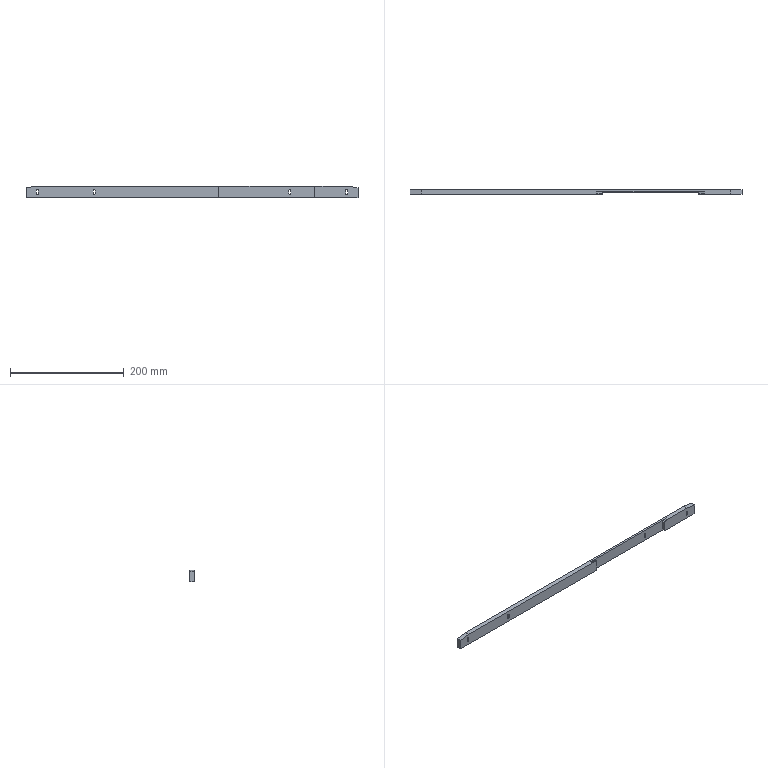Component | SolidWorks | SL010-LeftStreamline-1-1_SL010-02047858StopBarNo.4-1-2 | 1 solid | 32 faces | box 584 x 8 x 21 mm | volume 82637 mm3 | plane 24 | cylinder 8 | commonest cylinder face diameters 3.2 x8 | material White POM
build123d program:
from build123d import *

# Parameters (mm, degrees)
SKETCH1_2_W          = 584
SKETCH1_2_H          = 21
BOSS_EXTRUDE1_DEPTH  = 8
CUT_EXTRUDE1_2_DEPTH = 293.298
CHAMFER1_SIZE        = 3
CHAMFER1_SIZE2       = 20
CHAMFER2_SIZE        = 20
CHAMFER2_SIZE2       = 3
SKETCH4_W            = 169.5
SKETCH4_H            = 3.139
CUT_EXTRUDE3_DEPTH   = 293.863
CHAMFER3_SIZE        = 10
CHAMFER3_SIZE2       = 2.679
SKETCH1_W            = 169.5
SKETCH1_H            = 1.7
CUT_EXTRUDE1_DEPTH   = 293.863


with BuildPart() as part:
    # Sketch1_2 → Boss-Extrude1 (new body)
    with BuildSketch(Plane.XY):
        Rectangle(SKETCH1_2_W, SKETCH1_2_H)
    extrude(amount=BOSS_EXTRUDE1_DEPTH)

    # Sketch2 → Cut-Extrude1_2 (cut, through all)
    with BuildSketch(Plane.XY.offset(8)):
        with BuildLine():
            Line((173.6, 2.5), (173.6, -2.5))
            ThreePointArc((173.6, -2.5), (172, -4.1), (170.4, -2.5))
            Line((170.4, -2.5), (170.4, 2.5))
            ThreePointArc((170.4, 2.5), (172, 4.1), (173.6, 2.5))
        make_face()
        with BuildLine():
            Line((-273.6, 2.5), (-273.6, -2.5))
            ThreePointArc((-273.6, -2.5), (-272, -4.1), (-270.4, -2.5))
            Line((-270.4, -2.5), (-270.4, 2.5))
            ThreePointArc((-270.4, 2.5), (-272, 4.1), (-273.6, 2.5))
        make_face()
        with BuildLine():
            Line((273.6, 2.5), (273.6, -2.5))
            ThreePointArc((273.6, -2.5), (272, -4.1), (270.4, -2.5))
            Line((270.4, -2.5), (270.4, 2.5))
            ThreePointArc((270.4, 2.5), (272, 4.1), (273.6, 2.5))
        make_face()
        with BuildLine():
            Line((-173.6, 2.5), (-173.6, -2.5))
            ThreePointArc((-173.6, -2.5), (-172, -4.1), (-170.4, -2.5))
            Line((-170.4, -2.5), (-170.4, 2.5))
            ThreePointArc((-170.4, 2.5), (-172, 4.1), (-173.6, 2.5))
        make_face()
    extrude(amount=-CUT_EXTRUDE1_2_DEPTH, mode=Mode.SUBTRACT)

    # Chamfer1
    chamfer1_edges = [part.edges().sort_by_distance(p)[0] for p in [
        (292, 10.5, 4),
    ]]
    chamfer1_side = [part.faces().sort_by_distance(p)[0] for p in [
        (292, 0, 4),
    ]]
    chamfer(chamfer1_edges, length=CHAMFER1_SIZE, length2=CHAMFER1_SIZE2, reference=chamfer1_side[0])

    # Chamfer2
    chamfer2_edges = [part.edges().sort_by_distance(p)[0] for p in [
        (-292, 10.5, 4),
    ]]
    chamfer2_side = [part.faces().sort_by_distance(p)[0] for p in [
        (-10, 10.5, 4),
    ]]
    chamfer(chamfer2_edges, length=CHAMFER2_SIZE, length2=CHAMFER2_SIZE2, reference=chamfer2_side[0])

    # Sketch4 → Cut-Extrude3 (cut, through all)
    with BuildSketch(Plane.XZ.offset(10.5)):
        with Locations((-131.25, 2.431)):
            Rectangle(SKETCH4_W, SKETCH4_H)
    extrude(amount=-CUT_EXTRUDE3_DEPTH, mode=Mode.SUBTRACT)

    # Chamfer3
    chamfer3_edges = [part.edges().sort_by_distance(p)[0] for p in [
        (-216, 10.5, 2.431),
        (-46.5, 10.5, 2.431),
    ]]
    chamfer3_side = [part.faces().sort_by_distance(p)[0] for p in [
        (18.28, 10.5, 4.219),
    ]]
    chamfer(chamfer3_edges, length=CHAMFER3_SIZE, length2=CHAMFER3_SIZE2, reference=chamfer3_side[0])

    # Sketch1 → Cut-Extrude1 (cut, through all)
    with BuildSketch(Plane.XZ.offset(10.5)):
        with Locations((-131.25, 0.35)):
            Rectangle(SKETCH1_W, SKETCH1_H)
    extrude(amount=-CUT_EXTRUDE1_DEPTH, mode=Mode.SUBTRACT)


solid = part.part

# Placed as in the assembly
solid = solid.moved(Location((0, -109.904, -647.535), (-90, 0, 180)))
STEP:
#1=COLOUR_RGB('',0.7922,0.8196,0.9333);
#2=FILL_AREA_STYLE_COLOUR('',#1);
#3=FILL_AREA_STYLE('',(#2));
#4=SURFACE_STYLE_FILL_AREA(#3);
#5=SURFACE_SIDE_STYLE('',(#4));
#6=SURFACE_STYLE_USAGE(.BOTH.,#5);
#7=PRESENTATION_STYLE_ASSIGNMENT((#6));
#8=CARTESIAN_POINT('',(1.831,-4.327,-25.907));
#9=VERTEX_POINT('',#8);
#10=CARTESIAN_POINT('',(1.831,-4.169,-25.907));
#11=VERTEX_POINT('',#10);
#12=CARTESIAN_POINT('',(1.831,-4.293,-25.907));
#13=DIRECTION('',(0.,1.,0.));
#14=VECTOR('',#13,39.37);
#15=LINE('',#12,#14);
#16=EDGE_CURVE('',#9,#11,#15,.T.);
#17=ORIENTED_EDGE('',*,*,#16,.F.);
#18=CARTESIAN_POINT('',(-11.496,-4.327,-25.907));
#19=VERTEX_POINT('',#18);
#20=CARTESIAN_POINT('',(11.496,-4.327,-25.907));
#21=DIRECTION('',(-1.,0.,-0.));
#22=VECTOR('',#21,39.37);
#23=LINE('',#20,#22);
#24=EDGE_CURVE('',#9,#19,#23,.T.);
#25=ORIENTED_EDGE('',*,*,#24,.T.);
#26=CARTESIAN_POINT('',(-11.496,-4.012,-25.907));
#27=VERTEX_POINT('',#26);
#28=CARTESIAN_POINT('',(-11.496,-4.012,-25.907));
#29=DIRECTION('',(-0.,-1.,-0.));
#30=VECTOR('',#29,39.37);
#31=LINE('',#28,#30);
#32=EDGE_CURVE('',#27,#19,#31,.T.);
#33=ORIENTED_EDGE('',*,*,#32,.F.);
#34=CARTESIAN_POINT('',(11.496,-4.012,-25.907));
#35=VERTEX_POINT('',#34);
#36=CARTESIAN_POINT('',(11.496,-4.012,-25.907));
#37=DIRECTION('',(-1.,0.,-0.));
#38=VECTOR('',#37,39.37);
#39=LINE('',#36,#38);
#40=EDGE_CURVE('',#35,#27,#39,.T.);
#41=ORIENTED_EDGE('',*,*,#40,.F.);
#42=CARTESIAN_POINT('',(11.496,-4.327,-25.907));
#43=VERTEX_POINT('',#42);
#44=CARTESIAN_POINT('',(11.496,-4.012,-25.907));
#45=DIRECTION('',(-0.,-1.,-0.));
#46=VECTOR('',#45,39.37);
#47=LINE('',#44,#46);
#48=EDGE_CURVE('',#35,#43,#47,.T.);
#49=ORIENTED_EDGE('',*,*,#48,.T.);
#50=CARTESIAN_POINT('',(8.504,-4.327,-25.907));
#51=VERTEX_POINT('',#50);
#52=CARTESIAN_POINT('',(11.496,-4.327,-25.907));
#53=DIRECTION('',(-1.,0.,-0.));
#54=VECTOR('',#53,39.37);
#55=LINE('',#52,#54);
#56=EDGE_CURVE('',#43,#51,#55,.T.);
#57=ORIENTED_EDGE('',*,*,#56,.T.);
#58=CARTESIAN_POINT('',(8.504,-4.169,-25.907));
#59=VERTEX_POINT('',#58);
#60=CARTESIAN_POINT('',(8.504,-4.293,-25.907));
#61=DIRECTION('',(-0.,-1.,-0.));
#62=VECTOR('',#61,39.37);
#63=LINE('',#60,#62);
#64=EDGE_CURVE('',#59,#51,#63,.T.);
#65=ORIENTED_EDGE('',*,*,#64,.F.);
#66=CARTESIAN_POINT('',(1.831,-4.169,-25.907));
#67=DIRECTION('',(1.,-0.,0.));
#68=VECTOR('',#67,39.37);
#69=LINE('',#66,#68);
#70=EDGE_CURVE('',#11,#59,#69,.T.);
#71=ORIENTED_EDGE('',*,*,#70,.F.);
#72=EDGE_LOOP('',(#17,#25,#33,#41,#49,#57,#65,#71));
#73=FACE_OUTER_BOUND('',#72,.T.);
#74=CARTESIAN_POINT('',(11.496,-4.012,-25.907));
#75=DIRECTION('',(-0.,-0.,1.));
#76=DIRECTION('',(0.,1.,0.));
#77=AXIS2_PLACEMENT_3D('',#74,#75,#76);
#78=PLANE('',#77);
#79=ADVANCED_FACE('',(#73),#78,.F.);
#80=CARTESIAN_POINT('',(-6.835,-4.327,-25.592));
#81=VERTEX_POINT('',#80);
#82=CARTESIAN_POINT('',(-6.835,-4.327,-25.395));
#83=VERTEX_POINT('',#82);
#84=CARTESIAN_POINT('',(-6.835,-4.327,-25.395));
#85=DIRECTION('',(-0.,-0.,1.));
#86=VECTOR('',#85,39.37);
#87=LINE('',#84,#86);
#88=EDGE_CURVE('',#81,#83,#87,.T.);
#89=ORIENTED_EDGE('',*,*,#88,.T.);
#90=CARTESIAN_POINT('',(-6.709,-4.327,-25.395));
#91=VERTEX_POINT('',#90);
#92=CARTESIAN_POINT('',(-6.772,-4.327,-25.395));
#93=DIRECTION('',(0.,1.,0.));
#94=DIRECTION('',(-1.,0.,0.));
#95=AXIS2_PLACEMENT_3D('',#92,#93,#94);
#96=CIRCLE('',#95,0.06299);
#97=EDGE_CURVE('',#83,#91,#96,.T.);
#98=ORIENTED_EDGE('',*,*,#97,.T.);
#99=CARTESIAN_POINT('',(-6.709,-4.327,-25.592));
#100=VERTEX_POINT('',#99);
#101=CARTESIAN_POINT('',(-6.709,-4.327,-25.395));
#102=DIRECTION('',(0.,0.,-1.));
#103=VECTOR('',#102,39.37);
#104=LINE('',#101,#103);
#105=EDGE_CURVE('',#91,#100,#104,.T.);
#106=ORIENTED_EDGE('',*,*,#105,.T.);
#107=CARTESIAN_POINT('',(-6.772,-4.327,-25.592));
#108=DIRECTION('',(0.,1.,0.));
#109=DIRECTION('',(-1.,0.,0.));
#110=AXIS2_PLACEMENT_3D('',#107,#108,#109);
#111=CIRCLE('',#110,0.06299);
#112=EDGE_CURVE('',#100,#81,#111,.T.);
#113=ORIENTED_EDGE('',*,*,#112,.T.);
#114=EDGE_LOOP('',(#89,#98,#106,#113));
#115=FACE_BOUND('',#114,.T.);
#116=CARTESIAN_POINT('',(-10.772,-4.327,-25.592));
#117=VERTEX_POINT('',#116);
#118=CARTESIAN_POINT('',(-10.772,-4.327,-25.395));
#119=VERTEX_POINT('',#118);
#120=CARTESIAN_POINT('',(-10.772,-4.327,-25.395));
#121=DIRECTION('',(-0.,-0.,1.));
#122=VECTOR('',#121,39.37);
#123=LINE('',#120,#122);
#124=EDGE_CURVE('',#117,#119,#123,.T.);
#125=ORIENTED_EDGE('',*,*,#124,.T.);
#126=CARTESIAN_POINT('',(-10.646,-4.327,-25.395));
#127=VERTEX_POINT('',#126);
#128=CARTESIAN_POINT('',(-10.709,-4.327,-25.395));
#129=DIRECTION('',(0.,1.,0.));
#130=DIRECTION('',(-1.,0.,0.));
#131=AXIS2_PLACEMENT_3D('',#128,#129,#130);
#132=CIRCLE('',#131,0.06299);
#133=EDGE_CURVE('',#119,#127,#132,.T.);
#134=ORIENTED_EDGE('',*,*,#133,.T.);
#135=CARTESIAN_POINT('',(-10.646,-4.327,-25.592));
#136=VERTEX_POINT('',#135);
#137=CARTESIAN_POINT('',(-10.646,-4.327,-25.395));
#138=DIRECTION('',(0.,0.,-1.));
#139=VECTOR('',#138,39.37);
#140=LINE('',#137,#139);
#141=EDGE_CURVE('',#127,#136,#140,.T.);
#142=ORIENTED_EDGE('',*,*,#141,.T.);
#143=CARTESIAN_POINT('',(-10.709,-4.327,-25.592));
#144=DIRECTION('',(0.,1.,0.));
#145=DIRECTION('',(-1.,0.,0.));
#146=AXIS2_PLACEMENT_3D('',#143,#144,#145);
#147=CIRCLE('',#146,0.06299);
#148=EDGE_CURVE('',#136,#117,#147,.T.);
#149=ORIENTED_EDGE('',*,*,#148,.T.);
#150=EDGE_LOOP('',(#125,#134,#142,#149));
#151=FACE_BOUND('',#150,.T.);
#152=ORIENTED_EDGE('',*,*,#24,.F.);
#153=CARTESIAN_POINT('',(1.831,-4.327,-25.08));
#154=VERTEX_POINT('',#153);
#155=CARTESIAN_POINT('',(1.831,-4.327,-25.494));
#156=DIRECTION('',(-0.,-0.,1.));
#157=VECTOR('',#156,39.37);
#158=LINE('',#155,#157);
#159=EDGE_CURVE('',#9,#154,#158,.T.);
#160=ORIENTED_EDGE('',*,*,#159,.T.);
#161=CARTESIAN_POINT('',(-10.709,-4.327,-25.08));
#162=VERTEX_POINT('',#161);
#163=CARTESIAN_POINT('',(11.496,-4.327,-25.08));
#164=DIRECTION('',(1.,-0.,0.));
#165=VECTOR('',#164,39.37);
#166=LINE('',#163,#165);
#167=EDGE_CURVE('',#162,#154,#166,.T.);
#168=ORIENTED_EDGE('',*,*,#167,.F.);
#169=CARTESIAN_POINT('',(-11.496,-4.327,-25.198));
#170=VERTEX_POINT('',#169);
#171=CARTESIAN_POINT('',(-10.709,-4.327,-25.08));
#172=DIRECTION('',(-0.9889,0.,-0.1483));
#173=VECTOR('',#172,39.37);
#174=LINE('',#171,#173);
#175=EDGE_CURVE('',#162,#170,#174,.T.);
#176=ORIENTED_EDGE('',*,*,#175,.T.);
#177=CARTESIAN_POINT('',(-11.496,-4.327,-25.08));
#178=DIRECTION('',(-0.,-0.,1.));
#179=VECTOR('',#178,39.37);
#180=LINE('',#177,#179);
#181=EDGE_CURVE('',#19,#170,#180,.T.);
#182=ORIENTED_EDGE('',*,*,#181,.F.);
#183=EDGE_LOOP('',(#152,#160,#168,#176,#182));
#184=FACE_OUTER_BOUND('',#183,.T.);
#185=CARTESIAN_POINT('',(-0.,-4.327,-25.494));
#186=DIRECTION('',(0.,1.,0.));
#187=DIRECTION('',(-1.,0.,-0.));
#188=AXIS2_PLACEMENT_3D('',#185,#186,#187);
#189=PLANE('',#188);
#190=ADVANCED_FACE('',(#115,#151,#184),#189,.F.);
#191=CARTESIAN_POINT('',(1.831,-4.293,-25.08));
#192=VERTEX_POINT('',#191);
#193=CARTESIAN_POINT('',(1.437,-4.293,-25.08));
#194=VERTEX_POINT('',#193);
#195=CARTESIAN_POINT('',(1.831,-4.293,-25.08));
#196=DIRECTION('',(-1.,0.,-0.));
#197=VECTOR('',#196,39.37);
#198=LINE('',#195,#197);
#199=EDGE_CURVE('',#192,#194,#198,.T.);
#200=ORIENTED_EDGE('',*,*,#199,.F.);
#201=CARTESIAN_POINT('',(1.831,-4.293,-25.186));
#202=VERTEX_POINT('',#201);
#203=CARTESIAN_POINT('',(1.831,-4.293,-25.08));
#204=DIRECTION('',(0.,0.,-1.));
#205=VECTOR('',#204,39.37);
#206=LINE('',#203,#205);
#207=EDGE_CURVE('',#192,#202,#206,.T.);
#208=ORIENTED_EDGE('',*,*,#207,.T.);
#209=CARTESIAN_POINT('',(1.804,-4.293,-25.179));
#210=DIRECTION('',(-0.9659,0.,0.2588));
#211=VECTOR('',#210,39.37);
#212=LINE('',#209,#211);
#213=EDGE_CURVE('',#202,#194,#212,.T.);
#214=ORIENTED_EDGE('',*,*,#213,.T.);
#215=EDGE_LOOP('',(#200,#208,#214));
#216=FACE_OUTER_BOUND('',#215,.T.);
#217=CARTESIAN_POINT('',(1.831,-4.293,-25.08));
#218=DIRECTION('',(-0.,-1.,-0.));
#219=DIRECTION('',(1.,-0.,0.));
#220=AXIS2_PLACEMENT_3D('',#217,#218,#219);
#221=PLANE('',#220);
#222=ADVANCED_FACE('',(#216),#221,.F.);
#223=CARTESIAN_POINT('',(6.835,-4.169,-25.395));
#224=VERTEX_POINT('',#223);
#225=CARTESIAN_POINT('',(6.835,-4.012,-25.395));
#226=VERTEX_POINT('',#225);
#227=CARTESIAN_POINT('',(6.835,-4.327,-25.395));
#228=DIRECTION('',(0.,1.,0.));
#229=VECTOR('',#228,39.37);
#230=LINE('',#227,#229);
#231=EDGE_CURVE('',#224,#226,#230,.T.);
#232=ORIENTED_EDGE('',*,*,#231,.F.);
#233=CARTESIAN_POINT('',(6.709,-4.169,-25.395));
#234=VERTEX_POINT('',#233);
#235=CARTESIAN_POINT('',(6.772,-4.169,-25.395));
#236=DIRECTION('',(-0.,-1.,-0.));
#237=DIRECTION('',(-1.,0.,0.));
#238=AXIS2_PLACEMENT_3D('',#235,#236,#237);
#239=CIRCLE('',#238,0.06299);
#240=EDGE_CURVE('',#224,#234,#239,.T.);
#241=ORIENTED_EDGE('',*,*,#240,.T.);
#242=CARTESIAN_POINT('',(6.709,-4.012,-25.395));
#243=VERTEX_POINT('',#242);
#244=CARTESIAN_POINT('',(6.709,-4.327,-25.395));
#245=DIRECTION('',(0.,1.,0.));
#246=VECTOR('',#245,39.37);
#247=LINE('',#244,#246);
#248=EDGE_CURVE('',#234,#243,#247,.T.);
#249=ORIENTED_EDGE('',*,*,#248,.T.);
#250=CARTESIAN_POINT('',(6.772,-4.012,-25.395));
#251=DIRECTION('',(0.,1.,0.));
#252=DIRECTION('',(1.,0.,0.));
#253=AXIS2_PLACEMENT_3D('',#250,#251,#252);
#254=CIRCLE('',#253,0.06299);
#255=EDGE_CURVE('',#243,#226,#254,.T.);
#256=ORIENTED_EDGE('',*,*,#255,.T.);
#257=EDGE_LOOP('',(#232,#241,#249,#256));
#258=FACE_OUTER_BOUND('',#257,.T.);
#259=CARTESIAN_POINT('',(6.772,-4.327,-25.395));
#260=DIRECTION('',(0.,1.,0.));
#261=DIRECTION('',(-1.,0.,0.));
#262=AXIS2_PLACEMENT_3D('',#259,#260,#261);
#263=CYLINDRICAL_SURFACE('',#262,0.06299);
#264=ADVANCED_FACE('',(#258),#263,.F.);
#265=ORIENTED_EDGE('',*,*,#248,.F.);
#266=CARTESIAN_POINT('',(6.709,-4.169,-25.592));
#267=VERTEX_POINT('',#266);
#268=CARTESIAN_POINT('',(6.709,-4.169,-25.395));
#269=DIRECTION('',(0.,0.,-1.));
#270=VECTOR('',#269,39.37);
#271=LINE('',#268,#270);
#272=EDGE_CURVE('',#234,#267,#271,.T.);
#273=ORIENTED_EDGE('',*,*,#272,.T.);
#274=CARTESIAN_POINT('',(6.709,-4.012,-25.592));
#275=VERTEX_POINT('',#274);
#276=CARTESIAN_POINT('',(6.709,-4.327,-25.592));
#277=DIRECTION('',(0.,1.,0.));
#278=VECTOR('',#277,39.37);
#279=LINE('',#276,#278);
#280=EDGE_CURVE('',#267,#275,#279,.T.);
#281=ORIENTED_EDGE('',*,*,#280,.T.);
#282=CARTESIAN_POINT('',(6.709,-4.012,-25.395));
#283=DIRECTION('',(-0.,-0.,1.));
#284=VECTOR('',#283,39.37);
#285=LINE('',#282,#284);
#286=EDGE_CURVE('',#275,#243,#285,.T.);
#287=ORIENTED_EDGE('',*,*,#286,.T.);
#288=EDGE_LOOP('',(#265,#273,#281,#287));
#289=FACE_OUTER_BOUND('',#288,.T.);
#290=CARTESIAN_POINT('',(6.709,-4.327,-25.395));
#291=DIRECTION('',(-1.,0.,-0.));
#292=DIRECTION('',(-0.,-1.,-0.));
#293=AXIS2_PLACEMENT_3D('',#290,#291,#292);
#294=PLANE('',#293);
#295=ADVANCED_FACE('',(#289),#294,.F.);
#296=ORIENTED_EDGE('',*,*,#280,.F.);
#297=CARTESIAN_POINT('',(6.835,-4.169,-25.592));
#298=VERTEX_POINT('',#297);
#299=CARTESIAN_POINT('',(6.772,-4.169,-25.592));
#300=DIRECTION('',(-0.,-1.,-0.));
#301=DIRECTION('',(-1.,0.,0.));
#302=AXIS2_PLACEMENT_3D('',#299,#300,#301);
#303=CIRCLE('',#302,0.06299);
#304=EDGE_CURVE('',#267,#298,#303,.T.);
#305=ORIENTED_EDGE('',*,*,#304,.T.);
#306=CARTESIAN_POINT('',(6.835,-4.012,-25.592));
#307=VERTEX_POINT('',#306);
#308=CARTESIAN_POINT('',(6.835,-4.327,-25.592));
#309=DIRECTION('',(0.,1.,0.));
#310=VECTOR('',#309,39.37);
#311=LINE('',#308,#310);
#312=EDGE_CURVE('',#298,#307,#311,.T.);
#313=ORIENTED_EDGE('',*,*,#312,.T.);
#314=CARTESIAN_POINT('',(6.772,-4.012,-25.592));
#315=DIRECTION('',(0.,1.,0.));
#316=DIRECTION('',(1.,0.,0.));
#317=AXIS2_PLACEMENT_3D('',#314,#315,#316);
#318=CIRCLE('',#317,0.06299);
#319=EDGE_CURVE('',#307,#275,#318,.T.);
#320=ORIENTED_EDGE('',*,*,#319,.T.);
#321=EDGE_LOOP('',(#296,#305,#313,#320));
#322=FACE_OUTER_BOUND('',#321,.T.);
#323=CARTESIAN_POINT('',(6.772,-4.327,-25.592));
#324=DIRECTION('',(0.,1.,0.));
#325=DIRECTION('',(-1.,0.,0.));
#326=AXIS2_PLACEMENT_3D('',#323,#324,#325);
#327=CYLINDRICAL_SURFACE('',#326,0.06299);
#328=ADVANCED_FACE('',(#322),#327,.F.);
#329=ORIENTED_EDGE('',*,*,#312,.F.);
#330=CARTESIAN_POINT('',(6.835,-4.169,-25.395));
#331=DIRECTION('',(-0.,-0.,1.));
#332=VECTOR('',#331,39.37);
#333=LINE('',#330,#332);
#334=EDGE_CURVE('',#298,#224,#333,.T.);
#335=ORIENTED_EDGE('',*,*,#334,.T.);
#336=ORIENTED_EDGE('',*,*,#231,.T.);
#337=CARTESIAN_POINT('',(6.835,-4.012,-25.395));
#338=DIRECTION('',(0.,0.,-1.));
#339=VECTOR('',#338,39.37);
#340=LINE('',#337,#339);
#341=EDGE_CURVE('',#226,#307,#340,.T.);
#342=ORIENTED_EDGE('',*,*,#341,.T.);
#343=EDGE_LOOP('',(#329,#335,#336,#342));
#344=FACE_OUTER_BOUND('',#343,.T.);
#345=CARTESIAN_POINT('',(6.835,-4.327,-25.395));
#346=DIRECTION('',(1.,-0.,0.));
#347=DIRECTION('',(0.,1.,0.));
#348=AXIS2_PLACEMENT_3D('',#345,#346,#347);
#349=PLANE('',#348);
#350=ADVANCED_FACE('',(#344),#349,.F.);
#351=ORIENTED_EDGE('',*,*,#181,.T.);
#352=CARTESIAN_POINT('',(-11.496,-4.012,-25.198));
#353=VERTEX_POINT('',#352);
#354=CARTESIAN_POINT('',(-11.496,-4.012,-25.198));
#355=DIRECTION('',(0.,1.,0.));
#356=VECTOR('',#355,39.37);
#357=LINE('',#354,#356);
#358=EDGE_CURVE('',#170,#353,#357,.T.);
#359=ORIENTED_EDGE('',*,*,#358,.T.);
#360=CARTESIAN_POINT('',(-11.496,-4.012,-25.08));
#361=DIRECTION('',(-0.,-0.,1.));
#362=VECTOR('',#361,39.37);
#363=LINE('',#360,#362);
#364=EDGE_CURVE('',#27,#353,#363,.T.);
#365=ORIENTED_EDGE('',*,*,#364,.F.);
#366=ORIENTED_EDGE('',*,*,#32,.T.);
#367=EDGE_LOOP('',(#351,#359,#365,#366));
#368=FACE_OUTER_BOUND('',#367,.T.);
#369=CARTESIAN_POINT('',(-11.496,-4.012,-25.08));
#370=DIRECTION('',(1.,-0.,0.));
#371=DIRECTION('',(0.,1.,0.));
#372=AXIS2_PLACEMENT_3D('',#369,#370,#371);
#373=PLANE('',#372);
#374=ADVANCED_FACE('',(#368),#373,.F.);
#375=ORIENTED_EDGE('',*,*,#167,.T.);
#376=CARTESIAN_POINT('',(1.831,-4.347,-25.08));
#377=DIRECTION('',(0.,1.,0.));
#378=VECTOR('',#377,39.37);
#379=LINE('',#376,#378);
#380=EDGE_CURVE('',#154,#192,#379,.T.);
#381=ORIENTED_EDGE('',*,*,#380,.T.);
#382=ORIENTED_EDGE('',*,*,#199,.T.);
#383=CARTESIAN_POINT('',(1.437,-4.169,-25.08));
#384=VERTEX_POINT('',#383);
#385=CARTESIAN_POINT('',(1.437,-4.012,-25.08));
#386=DIRECTION('',(0.,1.,0.));
#387=VECTOR('',#386,39.37);
#388=LINE('',#385,#387);
#389=EDGE_CURVE('',#194,#384,#388,.T.);
#390=ORIENTED_EDGE('',*,*,#389,.T.);
#391=CARTESIAN_POINT('',(8.898,-4.169,-25.08));
#392=VERTEX_POINT('',#391);
#393=CARTESIAN_POINT('',(1.831,-4.169,-25.08));
#394=DIRECTION('',(1.,-0.,0.));
#395=VECTOR('',#394,39.37);
#396=LINE('',#393,#395);
#397=EDGE_CURVE('',#384,#392,#396,.T.);
#398=ORIENTED_EDGE('',*,*,#397,.T.);
#399=CARTESIAN_POINT('',(8.898,-4.293,-25.08));
#400=VERTEX_POINT('',#399);
#401=CARTESIAN_POINT('',(8.898,-4.012,-25.08));
#402=DIRECTION('',(-0.,-1.,-0.));
#403=VECTOR('',#402,39.37);
#404=LINE('',#401,#403);
#405=EDGE_CURVE('',#392,#400,#404,.T.);
#406=ORIENTED_EDGE('',*,*,#405,.T.);
#407=CARTESIAN_POINT('',(8.504,-4.293,-25.08));
#408=VERTEX_POINT('',#407);
#409=CARTESIAN_POINT('',(1.831,-4.293,-25.08));
#410=DIRECTION('',(-1.,0.,-0.));
#411=VECTOR('',#410,39.37);
#412=LINE('',#409,#411);
#413=EDGE_CURVE('',#400,#408,#412,.T.);
#414=ORIENTED_EDGE('',*,*,#413,.T.);
#415=CARTESIAN_POINT('',(8.504,-4.327,-25.08));
#416=VERTEX_POINT('',#415);
#417=CARTESIAN_POINT('',(8.504,-4.347,-25.08));
#418=DIRECTION('',(-0.,-1.,-0.));
#419=VECTOR('',#418,39.37);
#420=LINE('',#417,#419);
#421=EDGE_CURVE('',#408,#416,#420,.T.);
#422=ORIENTED_EDGE('',*,*,#421,.T.);
#423=CARTESIAN_POINT('',(10.709,-4.327,-25.08));
#424=VERTEX_POINT('',#423);
#425=CARTESIAN_POINT('',(11.496,-4.327,-25.08));
#426=DIRECTION('',(1.,-0.,0.));
#427=VECTOR('',#426,39.37);
#428=LINE('',#425,#427);
#429=EDGE_CURVE('',#416,#424,#428,.T.);
#430=ORIENTED_EDGE('',*,*,#429,.T.);
#431=CARTESIAN_POINT('',(10.709,-4.012,-25.08));
#432=VERTEX_POINT('',#431);
#433=CARTESIAN_POINT('',(10.709,-4.012,-25.08));
#434=DIRECTION('',(0.,1.,0.));
#435=VECTOR('',#434,39.37);
#436=LINE('',#433,#435);
#437=EDGE_CURVE('',#424,#432,#436,.T.);
#438=ORIENTED_EDGE('',*,*,#437,.T.);
#439=CARTESIAN_POINT('',(-10.709,-4.012,-25.08));
#440=VERTEX_POINT('',#439);
#441=CARTESIAN_POINT('',(11.496,-4.012,-25.08));
#442=DIRECTION('',(1.,-0.,0.));
#443=VECTOR('',#442,39.37);
#444=LINE('',#441,#443);
#445=EDGE_CURVE('',#440,#432,#444,.T.);
#446=ORIENTED_EDGE('',*,*,#445,.F.);
#447=CARTESIAN_POINT('',(-10.709,-4.012,-25.08));
#448=DIRECTION('',(-0.,-1.,-0.));
#449=VECTOR('',#448,39.37);
#450=LINE('',#447,#449);
#451=EDGE_CURVE('',#440,#162,#450,.T.);
#452=ORIENTED_EDGE('',*,*,#451,.T.);
#453=EDGE_LOOP('',(#375,#381,#382,#390,#398,#406,#414,#422,#430,#438,#446,#452));
#454=FACE_OUTER_BOUND('',#453,.T.);
#455=CARTESIAN_POINT('',(11.496,-4.012,-25.08));
#456=DIRECTION('',(0.,0.,-1.));
#457=DIRECTION('',(-0.,-1.,-0.));
#458=AXIS2_PLACEMENT_3D('',#455,#456,#457);
#459=PLANE('',#458);
#460=ADVANCED_FACE('',(#454),#459,.F.);
#461=CARTESIAN_POINT('',(11.496,-4.012,-25.198));
#462=VERTEX_POINT('',#461);
#463=CARTESIAN_POINT('',(11.496,-4.012,-25.08));
#464=DIRECTION('',(0.,0.,-1.));
#465=VECTOR('',#464,39.37);
#466=LINE('',#463,#465);
#467=EDGE_CURVE('',#462,#35,#466,.T.);
#468=ORIENTED_EDGE('',*,*,#467,.F.);
#469=CARTESIAN_POINT('',(11.496,-4.327,-25.198));
#470=VERTEX_POINT('',#469);
#471=CARTESIAN_POINT('',(11.496,-4.012,-25.198));
#472=DIRECTION('',(-0.,-1.,-0.));
#473=VECTOR('',#472,39.37);
#474=LINE('',#471,#473);
#475=EDGE_CURVE('',#462,#470,#474,.T.);
#476=ORIENTED_EDGE('',*,*,#475,.T.);
#477=CARTESIAN_POINT('',(11.496,-4.327,-25.08));
#478=DIRECTION('',(0.,0.,-1.));
#479=VECTOR('',#478,39.37);
#480=LINE('',#477,#479);
#481=EDGE_CURVE('',#470,#43,#480,.T.);
#482=ORIENTED_EDGE('',*,*,#481,.T.);
#483=ORIENTED_EDGE('',*,*,#48,.F.);
#484=EDGE_LOOP('',(#468,#476,#482,#483));
#485=FACE_OUTER_BOUND('',#484,.T.);
#486=CARTESIAN_POINT('',(11.496,-4.012,-25.08));
#487=DIRECTION('',(-1.,0.,-0.));
#488=DIRECTION('',(-0.,-1.,-0.));
#489=AXIS2_PLACEMENT_3D('',#486,#487,#488);
#490=PLANE('',#489);
#491=ADVANCED_FACE('',(#485),#490,.F.);
#492=ORIENTED_EDGE('',*,*,#255,.F.);
#493=ORIENTED_EDGE('',*,*,#286,.F.);
#494=ORIENTED_EDGE('',*,*,#319,.F.);
#495=ORIENTED_EDGE('',*,*,#341,.F.);
#496=EDGE_LOOP('',(#492,#493,#494,#495));
#497=FACE_BOUND('',#496,.T.);
#498=CARTESIAN_POINT('',(-10.772,-4.012,-25.395));
#499=VERTEX_POINT('',#498);
#500=CARTESIAN_POINT('',(-10.646,-4.012,-25.395));
#501=VERTEX_POINT('',#500);
#502=CARTESIAN_POINT('',(-10.709,-4.012,-25.395));
#503=DIRECTION('',(0.,1.,0.));
#504=DIRECTION('',(-1.,0.,0.));
#505=AXIS2_PLACEMENT_3D('',#502,#503,#504);
#506=CIRCLE('',#505,0.06299);
#507=EDGE_CURVE('',#499,#501,#506,.T.);
#508=ORIENTED_EDGE('',*,*,#507,.F.);
#509=CARTESIAN_POINT('',(-10.772,-4.012,-25.592));
#510=VERTEX_POINT('',#509);
#511=CARTESIAN_POINT('',(-10.772,-4.012,-25.395));
#512=DIRECTION('',(-0.,-0.,1.));
#513=VECTOR('',#512,39.37);
#514=LINE('',#511,#513);
#515=EDGE_CURVE('',#510,#499,#514,.T.);
#516=ORIENTED_EDGE('',*,*,#515,.F.);
#517=CARTESIAN_POINT('',(-10.646,-4.012,-25.592));
#518=VERTEX_POINT('',#517);
#519=CARTESIAN_POINT('',(-10.709,-4.012,-25.592));
#520=DIRECTION('',(0.,1.,0.));
#521=DIRECTION('',(-1.,0.,0.));
#522=AXIS2_PLACEMENT_3D('',#519,#520,#521);
#523=CIRCLE('',#522,0.06299);
#524=EDGE_CURVE('',#518,#510,#523,.T.);
#525=ORIENTED_EDGE('',*,*,#524,.F.);
#526=CARTESIAN_POINT('',(-10.646,-4.012,-25.395));
#527=DIRECTION('',(0.,0.,-1.));
#528=VECTOR('',#527,39.37);
#529=LINE('',#526,#528);
#530=EDGE_CURVE('',#501,#518,#529,.T.);
#531=ORIENTED_EDGE('',*,*,#530,.F.);
#532=EDGE_LOOP('',(#508,#516,#525,#531));
#533=FACE_BOUND('',#532,.T.);
#534=CARTESIAN_POINT('',(10.646,-4.012,-25.395));
#535=VERTEX_POINT('',#534);
#536=CARTESIAN_POINT('',(10.772,-4.012,-25.395));
#537=VERTEX_POINT('',#536);
#538=CARTESIAN_POINT('',(10.709,-4.012,-25.395));
#539=DIRECTION('',(0.,1.,0.));
#540=DIRECTION('',(1.,0.,0.));
#541=AXIS2_PLACEMENT_3D('',#538,#539,#540);
#542=CIRCLE('',#541,0.06299);
#543=EDGE_CURVE('',#535,#537,#542,.T.);
#544=ORIENTED_EDGE('',*,*,#543,.F.);
#545=CARTESIAN_POINT('',(10.646,-4.012,-25.592));
#546=VERTEX_POINT('',#545);
#547=CARTESIAN_POINT('',(10.646,-4.012,-25.395));
#548=DIRECTION('',(-0.,-0.,1.));
#549=VECTOR('',#548,39.37);
#550=LINE('',#547,#549);
#551=EDGE_CURVE('',#546,#535,#550,.T.);
#552=ORIENTED_EDGE('',*,*,#551,.F.);
#553=CARTESIAN_POINT('',(10.772,-4.012,-25.592));
#554=VERTEX_POINT('',#553);
#555=CARTESIAN_POINT('',(10.709,-4.012,-25.592));
#556=DIRECTION('',(0.,1.,0.));
#557=DIRECTION('',(1.,0.,0.));
#558=AXIS2_PLACEMENT_3D('',#555,#556,#557);
#559=CIRCLE('',#558,0.06299);
#560=EDGE_CURVE('',#554,#546,#559,.T.);
#561=ORIENTED_EDGE('',*,*,#560,.F.);
#562=CARTESIAN_POINT('',(10.772,-4.012,-25.395));
#563=DIRECTION('',(0.,0.,-1.));
#564=VECTOR('',#563,39.37);
#565=LINE('',#562,#564);
#566=EDGE_CURVE('',#537,#554,#565,.T.);
#567=ORIENTED_EDGE('',*,*,#566,.F.);
#568=EDGE_LOOP('',(#544,#552,#561,#567));
#569=FACE_BOUND('',#568,.T.);
#570=CARTESIAN_POINT('',(-6.835,-4.012,-25.395));
#571=VERTEX_POINT('',#570);
#572=CARTESIAN_POINT('',(-6.709,-4.012,-25.395));
#573=VERTEX_POINT('',#572);
#574=CARTESIAN_POINT('',(-6.772,-4.012,-25.395));
#575=DIRECTION('',(0.,1.,0.));
#576=DIRECTION('',(-1.,0.,0.));
#577=AXIS2_PLACEMENT_3D('',#574,#575,#576);
#578=CIRCLE('',#577,0.06299);
#579=EDGE_CURVE('',#571,#573,#578,.T.);
#580=ORIENTED_EDGE('',*,*,#579,.F.);
#581=CARTESIAN_POINT('',(-6.835,-4.012,-25.592));
#582=VERTEX_POINT('',#581);
#583=CARTESIAN_POINT('',(-6.835,-4.012,-25.395));
#584=DIRECTION('',(-0.,-0.,1.));
#585=VECTOR('',#584,39.37);
#586=LINE('',#583,#585);
#587=EDGE_CURVE('',#582,#571,#586,.T.);
#588=ORIENTED_EDGE('',*,*,#587,.F.);
#589=CARTESIAN_POINT('',(-6.709,-4.012,-25.592));
#590=VERTEX_POINT('',#589);
#591=CARTESIAN_POINT('',(-6.772,-4.012,-25.592));
#592=DIRECTION('',(0.,1.,0.));
#593=DIRECTION('',(-1.,0.,0.));
#594=AXIS2_PLACEMENT_3D('',#591,#592,#593);
#595=CIRCLE('',#594,0.06299);
#596=EDGE_CURVE('',#590,#582,#595,.T.);
#597=ORIENTED_EDGE('',*,*,#596,.F.);
#598=CARTESIAN_POINT('',(-6.709,-4.012,-25.395));
#599=DIRECTION('',(0.,0.,-1.));
#600=VECTOR('',#599,39.37);
#601=LINE('',#598,#600);
#602=EDGE_CURVE('',#573,#590,#601,.T.);
#603=ORIENTED_EDGE('',*,*,#602,.F.);
#604=EDGE_LOOP('',(#580,#588,#597,#603));
#605=FACE_BOUND('',#604,.T.);
#606=ORIENTED_EDGE('',*,*,#445,.T.);
#607=CARTESIAN_POINT('',(0.2963,-4.012,-23.518));
#608=DIRECTION('',(0.9889,-0.,-0.1483));
#609=VECTOR('',#608,39.37);
#610=LINE('',#607,#609);
#611=EDGE_CURVE('',#432,#462,#610,.T.);
#612=ORIENTED_EDGE('',*,*,#611,.T.);
#613=ORIENTED_EDGE('',*,*,#467,.T.);
#614=ORIENTED_EDGE('',*,*,#40,.T.);
#615=ORIENTED_EDGE('',*,*,#364,.T.);
#616=CARTESIAN_POINT('',(-0.2963,-4.012,-23.518));
#617=DIRECTION('',(0.9889,-0.,0.1483));
#618=VECTOR('',#617,39.37);
#619=LINE('',#616,#618);
#620=EDGE_CURVE('',#353,#440,#619,.T.);
#621=ORIENTED_EDGE('',*,*,#620,.T.);
#622=EDGE_LOOP('',(#606,#612,#613,#614,#615,#621));
#623=FACE_OUTER_BOUND('',#622,.T.);
#624=CARTESIAN_POINT('',(-0.,-4.012,-25.494));
#625=DIRECTION('',(0.,1.,0.));
#626=DIRECTION('',(-1.,0.,-0.));
#627=AXIS2_PLACEMENT_3D('',#624,#625,#626);
#628=PLANE('',#627);
#629=ADVANCED_FACE('',(#497,#533,#569,#605,#623),#628,.T.);
#630=CARTESIAN_POINT('',(10.646,-4.327,-25.592));
#631=VERTEX_POINT('',#630);
#632=CARTESIAN_POINT('',(10.646,-4.327,-25.395));
#633=VERTEX_POINT('',#632);
#634=CARTESIAN_POINT('',(10.646,-4.327,-25.395));
#635=DIRECTION('',(-0.,-0.,1.));
#636=VECTOR('',#635,39.37);
#637=LINE('',#634,#636);
#638=EDGE_CURVE('',#631,#633,#637,.T.);
#639=ORIENTED_EDGE('',*,*,#638,.T.);
#640=CARTESIAN_POINT('',(10.772,-4.327,-25.395));
#641=VERTEX_POINT('',#640);
#642=CARTESIAN_POINT('',(10.709,-4.327,-25.395));
#643=DIRECTION('',(0.,1.,0.));
#644=DIRECTION('',(1.,0.,0.));
#645=AXIS2_PLACEMENT_3D('',#642,#643,#644);
#646=CIRCLE('',#645,0.06299);
#647=EDGE_CURVE('',#633,#641,#646,.T.);
#648=ORIENTED_EDGE('',*,*,#647,.T.);
#649=CARTESIAN_POINT('',(10.772,-4.327,-25.592));
#650=VERTEX_POINT('',#649);
#651=CARTESIAN_POINT('',(10.772,-4.327,-25.395));
#652=DIRECTION('',(0.,0.,-1.));
#653=VECTOR('',#652,39.37);
#654=LINE('',#651,#653);
#655=EDGE_CURVE('',#641,#650,#654,.T.);
#656=ORIENTED_EDGE('',*,*,#655,.T.);
#657=CARTESIAN_POINT('',(10.709,-4.327,-25.592));
#658=DIRECTION('',(0.,1.,0.));
#659=DIRECTION('',(1.,0.,0.));
#660=AXIS2_PLACEMENT_3D('',#657,#658,#659);
#661=CIRCLE('',#660,0.06299);
#662=EDGE_CURVE('',#650,#631,#661,.T.);
#663=ORIENTED_EDGE('',*,*,#662,.T.);
#664=EDGE_LOOP('',(#639,#648,#656,#663));
#665=FACE_BOUND('',#664,.T.);
#666=ORIENTED_EDGE('',*,*,#429,.F.);
#667=CARTESIAN_POINT('',(8.504,-4.327,-25.494));
#668=DIRECTION('',(0.,0.,-1.));
#669=VECTOR('',#668,39.37);
#670=LINE('',#667,#669);
#671=EDGE_CURVE('',#416,#51,#670,.T.);
#672=ORIENTED_EDGE('',*,*,#671,.T.);
#673=ORIENTED_EDGE('',*,*,#56,.F.);
#674=ORIENTED_EDGE('',*,*,#481,.F.);
#675=CARTESIAN_POINT('',(11.496,-4.327,-25.198));
#676=DIRECTION('',(-0.9889,0.,0.1483));
#677=VECTOR('',#676,39.37);
#678=LINE('',#675,#677);
#679=EDGE_CURVE('',#470,#424,#678,.T.);
#680=ORIENTED_EDGE('',*,*,#679,.T.);
#681=EDGE_LOOP('',(#666,#672,#673,#674,#680));
#682=FACE_OUTER_BOUND('',#681,.T.);
#683=CARTESIAN_POINT('',(-0.,-4.327,-25.494));
#684=DIRECTION('',(0.,1.,0.));
#685=DIRECTION('',(-1.,0.,-0.));
#686=AXIS2_PLACEMENT_3D('',#683,#684,#685);
#687=PLANE('',#686);
#688=ADVANCED_FACE('',(#665,#682),#687,.F.);
#689=ORIENTED_EDGE('',*,*,#579,.T.);
#690=CARTESIAN_POINT('',(-6.709,-4.327,-25.395));
#691=DIRECTION('',(0.,1.,0.));
#692=VECTOR('',#691,39.37);
#693=LINE('',#690,#692);
#694=EDGE_CURVE('',#91,#573,#693,.T.);
#695=ORIENTED_EDGE('',*,*,#694,.F.);
#696=ORIENTED_EDGE('',*,*,#97,.F.);
#697=CARTESIAN_POINT('',(-6.835,-4.327,-25.395));
#698=DIRECTION('',(0.,1.,0.));
#699=VECTOR('',#698,39.37);
#700=LINE('',#697,#699);
#701=EDGE_CURVE('',#83,#571,#700,.T.);
#702=ORIENTED_EDGE('',*,*,#701,.T.);
#703=EDGE_LOOP('',(#689,#695,#696,#702));
#704=FACE_OUTER_BOUND('',#703,.T.);
#705=CARTESIAN_POINT('',(-6.772,-4.327,-25.395));
#706=DIRECTION('',(0.,1.,0.));
#707=DIRECTION('',(-1.,0.,0.));
#708=AXIS2_PLACEMENT_3D('',#705,#706,#707);
#709=CYLINDRICAL_SURFACE('',#708,0.06299);
#710=ADVANCED_FACE('',(#704),#709,.F.);
#711=ORIENTED_EDGE('',*,*,#587,.T.);
#712=ORIENTED_EDGE('',*,*,#701,.F.);
#713=ORIENTED_EDGE('',*,*,#88,.F.);
#714=CARTESIAN_POINT('',(-6.835,-4.327,-25.592));
#715=DIRECTION('',(0.,1.,0.));
#716=VECTOR('',#715,39.37);
#717=LINE('',#714,#716);
#718=EDGE_CURVE('',#81,#582,#717,.T.);
#719=ORIENTED_EDGE('',*,*,#718,.T.);
#720=EDGE_LOOP('',(#711,#712,#713,#719));
#721=FACE_OUTER_BOUND('',#720,.T.);
#722=CARTESIAN_POINT('',(-6.835,-4.327,-25.395));
#723=DIRECTION('',(-1.,0.,-0.));
#724=DIRECTION('',(-0.,-1.,-0.));
#725=AXIS2_PLACEMENT_3D('',#722,#723,#724);
#726=PLANE('',#725);
#727=ADVANCED_FACE('',(#721),#726,.F.);
#728=ORIENTED_EDGE('',*,*,#596,.T.);
#729=ORIENTED_EDGE('',*,*,#718,.F.);
#730=ORIENTED_EDGE('',*,*,#112,.F.);
#731=CARTESIAN_POINT('',(-6.709,-4.327,-25.592));
#732=DIRECTION('',(0.,1.,0.));
#733=VECTOR('',#732,39.37);
#734=LINE('',#731,#733);
#735=EDGE_CURVE('',#100,#590,#734,.T.);
#736=ORIENTED_EDGE('',*,*,#735,.T.);
#737=EDGE_LOOP('',(#728,#729,#730,#736));
#738=FACE_OUTER_BOUND('',#737,.T.);
#739=CARTESIAN_POINT('',(-6.772,-4.327,-25.592));
#740=DIRECTION('',(0.,1.,0.));
#741=DIRECTION('',(-1.,0.,0.));
#742=AXIS2_PLACEMENT_3D('',#739,#740,#741);
#743=CYLINDRICAL_SURFACE('',#742,0.06299);
#744=ADVANCED_FACE('',(#738),#743,.F.);
#745=ORIENTED_EDGE('',*,*,#602,.T.);
#746=ORIENTED_EDGE('',*,*,#735,.F.);
#747=ORIENTED_EDGE('',*,*,#105,.F.);
#748=ORIENTED_EDGE('',*,*,#694,.T.);
#749=EDGE_LOOP('',(#745,#746,#747,#748));
#750=FACE_OUTER_BOUND('',#749,.T.);
#751=CARTESIAN_POINT('',(-6.709,-4.327,-25.395));
#752=DIRECTION('',(1.,-0.,0.));
#753=DIRECTION('',(0.,1.,0.));
#754=AXIS2_PLACEMENT_3D('',#751,#752,#753);
#755=PLANE('',#754);
#756=ADVANCED_FACE('',(#750),#755,.F.);
#757=ORIENTED_EDGE('',*,*,#543,.T.);
#758=CARTESIAN_POINT('',(10.772,-4.327,-25.395));
#759=DIRECTION('',(0.,1.,0.));
#760=VECTOR('',#759,39.37);
#761=LINE('',#758,#760);
#762=EDGE_CURVE('',#641,#537,#761,.T.);
#763=ORIENTED_EDGE('',*,*,#762,.F.);
#764=ORIENTED_EDGE('',*,*,#647,.F.);
#765=CARTESIAN_POINT('',(10.646,-4.327,-25.395));
#766=DIRECTION('',(0.,1.,0.));
#767=VECTOR('',#766,39.37);
#768=LINE('',#765,#767);
#769=EDGE_CURVE('',#633,#535,#768,.T.);
#770=ORIENTED_EDGE('',*,*,#769,.T.);
#771=EDGE_LOOP('',(#757,#763,#764,#770));
#772=FACE_OUTER_BOUND('',#771,.T.);
#773=CARTESIAN_POINT('',(10.709,-4.327,-25.395));
#774=DIRECTION('',(0.,1.,0.));
#775=DIRECTION('',(-1.,0.,0.));
#776=AXIS2_PLACEMENT_3D('',#773,#774,#775);
#777=CYLINDRICAL_SURFACE('',#776,0.06299);
#778=ADVANCED_FACE('',(#772),#777,.F.);
#779=ORIENTED_EDGE('',*,*,#551,.T.);
#780=ORIENTED_EDGE('',*,*,#769,.F.);
#781=ORIENTED_EDGE('',*,*,#638,.F.);
#782=CARTESIAN_POINT('',(10.646,-4.327,-25.592));
#783=DIRECTION('',(0.,1.,0.));
#784=VECTOR('',#783,39.37);
#785=LINE('',#782,#784);
#786=EDGE_CURVE('',#631,#546,#785,.T.);
#787=ORIENTED_EDGE('',*,*,#786,.T.);
#788=EDGE_LOOP('',(#779,#780,#781,#787));
#789=FACE_OUTER_BOUND('',#788,.T.);
#790=CARTESIAN_POINT('',(10.646,-4.327,-25.395));
#791=DIRECTION('',(-1.,0.,-0.));
#792=DIRECTION('',(-0.,-1.,-0.));
#793=AXIS2_PLACEMENT_3D('',#790,#791,#792);
#794=PLANE('',#793);
#795=ADVANCED_FACE('',(#789),#794,.F.);
#796=ORIENTED_EDGE('',*,*,#560,.T.);
#797=ORIENTED_EDGE('',*,*,#786,.F.);
#798=ORIENTED_EDGE('',*,*,#662,.F.);
#799=CARTESIAN_POINT('',(10.772,-4.327,-25.592));
#800=DIRECTION('',(0.,1.,0.));
#801=VECTOR('',#800,39.37);
#802=LINE('',#799,#801);
#803=EDGE_CURVE('',#650,#554,#802,.T.);
#804=ORIENTED_EDGE('',*,*,#803,.T.);
#805=EDGE_LOOP('',(#796,#797,#798,#804));
#806=FACE_OUTER_BOUND('',#805,.T.);
#807=CARTESIAN_POINT('',(10.709,-4.327,-25.592));
#808=DIRECTION('',(0.,1.,0.));
#809=DIRECTION('',(-1.,0.,0.));
#810=AXIS2_PLACEMENT_3D('',#807,#808,#809);
#811=CYLINDRICAL_SURFACE('',#810,0.06299);
#812=ADVANCED_FACE('',(#806),#811,.F.);
#813=ORIENTED_EDGE('',*,*,#566,.T.);
#814=ORIENTED_EDGE('',*,*,#803,.F.);
#815=ORIENTED_EDGE('',*,*,#655,.F.);
#816=ORIENTED_EDGE('',*,*,#762,.T.);
#817=EDGE_LOOP('',(#813,#814,#815,#816));
#818=FACE_OUTER_BOUND('',#817,.T.);
#819=CARTESIAN_POINT('',(10.772,-4.327,-25.395));
#820=DIRECTION('',(1.,-0.,0.));
#821=DIRECTION('',(0.,1.,0.));
#822=AXIS2_PLACEMENT_3D('',#819,#820,#821);
#823=PLANE('',#822);
#824=ADVANCED_FACE('',(#818),#823,.F.);
#825=ORIENTED_EDGE('',*,*,#507,.T.);
#826=CARTESIAN_POINT('',(-10.646,-4.327,-25.395));
#827=DIRECTION('',(0.,1.,0.));
#828=VECTOR('',#827,39.37);
#829=LINE('',#826,#828);
#830=EDGE_CURVE('',#127,#501,#829,.T.);
#831=ORIENTED_EDGE('',*,*,#830,.F.);
#832=ORIENTED_EDGE('',*,*,#133,.F.);
#833=CARTESIAN_POINT('',(-10.772,-4.327,-25.395));
#834=DIRECTION('',(0.,1.,0.));
#835=VECTOR('',#834,39.37);
#836=LINE('',#833,#835);
#837=EDGE_CURVE('',#119,#499,#836,.T.);
#838=ORIENTED_EDGE('',*,*,#837,.T.);
#839=EDGE_LOOP('',(#825,#831,#832,#838));
#840=FACE_OUTER_BOUND('',#839,.T.);
#841=CARTESIAN_POINT('',(-10.709,-4.327,-25.395));
#842=DIRECTION('',(0.,1.,0.));
#843=DIRECTION('',(-1.,0.,0.));
#844=AXIS2_PLACEMENT_3D('',#841,#842,#843);
#845=CYLINDRICAL_SURFACE('',#844,0.06299);
#846=ADVANCED_FACE('',(#840),#845,.F.);
#847=ORIENTED_EDGE('',*,*,#515,.T.);
#848=ORIENTED_EDGE('',*,*,#837,.F.);
#849=ORIENTED_EDGE('',*,*,#124,.F.);
#850=CARTESIAN_POINT('',(-10.772,-4.327,-25.592));
#851=DIRECTION('',(0.,1.,0.));
#852=VECTOR('',#851,39.37);
#853=LINE('',#850,#852);
#854=EDGE_CURVE('',#117,#510,#853,.T.);
#855=ORIENTED_EDGE('',*,*,#854,.T.);
#856=EDGE_LOOP('',(#847,#848,#849,#855));
#857=FACE_OUTER_BOUND('',#856,.T.);
#858=CARTESIAN_POINT('',(-10.772,-4.327,-25.395));
#859=DIRECTION('',(-1.,0.,-0.));
#860=DIRECTION('',(-0.,-1.,-0.));
#861=AXIS2_PLACEMENT_3D('',#858,#859,#860);
#862=PLANE('',#861);
#863=ADVANCED_FACE('',(#857),#862,.F.);
#864=ORIENTED_EDGE('',*,*,#524,.T.);
#865=ORIENTED_EDGE('',*,*,#854,.F.);
#866=ORIENTED_EDGE('',*,*,#148,.F.);
#867=CARTESIAN_POINT('',(-10.646,-4.327,-25.592));
#868=DIRECTION('',(0.,1.,0.));
#869=VECTOR('',#868,39.37);
#870=LINE('',#867,#869);
#871=EDGE_CURVE('',#136,#518,#870,.T.);
#872=ORIENTED_EDGE('',*,*,#871,.T.);
#873=EDGE_LOOP('',(#864,#865,#866,#872));
#874=FACE_OUTER_BOUND('',#873,.T.);
#875=CARTESIAN_POINT('',(-10.709,-4.327,-25.592));
#876=DIRECTION('',(0.,1.,0.));
#877=DIRECTION('',(-1.,0.,0.));
#878=AXIS2_PLACEMENT_3D('',#875,#876,#877);
#879=CYLINDRICAL_SURFACE('',#878,0.06299);
#880=ADVANCED_FACE('',(#874),#879,.F.);
#881=ORIENTED_EDGE('',*,*,#530,.T.);
#882=ORIENTED_EDGE('',*,*,#871,.F.);
#883=ORIENTED_EDGE('',*,*,#141,.F.);
#884=ORIENTED_EDGE('',*,*,#830,.T.);
#885=EDGE_LOOP('',(#881,#882,#883,#884));
#886=FACE_OUTER_BOUND('',#885,.T.);
#887=CARTESIAN_POINT('',(-10.646,-4.327,-25.395));
#888=DIRECTION('',(1.,-0.,0.));
#889=DIRECTION('',(0.,1.,0.));
#890=AXIS2_PLACEMENT_3D('',#887,#888,#889);
#891=PLANE('',#890);
#892=ADVANCED_FACE('',(#886),#891,.F.);
#893=ORIENTED_EDGE('',*,*,#620,.F.);
#894=ORIENTED_EDGE('',*,*,#358,.F.);
#895=ORIENTED_EDGE('',*,*,#175,.F.);
#896=ORIENTED_EDGE('',*,*,#451,.F.);
#897=EDGE_LOOP('',(#893,#894,#895,#896));
#898=FACE_OUTER_BOUND('',#897,.T.);
#899=CARTESIAN_POINT('',(-10.709,-4.012,-25.08));
#900=DIRECTION('',(0.1483,0.,-0.9889));
#901=DIRECTION('',(-0.,-1.,-0.));
#902=AXIS2_PLACEMENT_3D('',#899,#900,#901);
#903=PLANE('',#902);
#904=ADVANCED_FACE('',(#898),#903,.F.);
#905=ORIENTED_EDGE('',*,*,#611,.F.);
#906=ORIENTED_EDGE('',*,*,#437,.F.);
#907=ORIENTED_EDGE('',*,*,#679,.F.);
#908=ORIENTED_EDGE('',*,*,#475,.F.);
#909=EDGE_LOOP('',(#905,#906,#907,#908));
#910=FACE_OUTER_BOUND('',#909,.T.);
#911=CARTESIAN_POINT('',(11.496,-4.012,-25.198));
#912=DIRECTION('',(-0.1483,0.,-0.9889));
#913=DIRECTION('',(-0.,-1.,-0.));
#914=AXIS2_PLACEMENT_3D('',#911,#912,#913);
#915=PLANE('',#914);
#916=ADVANCED_FACE('',(#910),#915,.F.);
#917=ORIENTED_EDGE('',*,*,#70,.T.);
#918=CARTESIAN_POINT('',(8.504,-4.169,-25.186));
#919=VERTEX_POINT('',#918);
#920=CARTESIAN_POINT('',(8.504,-4.169,-25.08));
#921=DIRECTION('',(0.,0.,-1.));
#922=VECTOR('',#921,39.37);
#923=LINE('',#920,#922);
#924=EDGE_CURVE('',#919,#59,#923,.T.);
#925=ORIENTED_EDGE('',*,*,#924,.F.);
#926=CARTESIAN_POINT('',(2.304,-4.169,-26.847));
#927=DIRECTION('',(0.9659,-0.,0.2588));
#928=VECTOR('',#927,39.37);
#929=LINE('',#926,#928);
#930=EDGE_CURVE('',#919,#392,#929,.T.);
#931=ORIENTED_EDGE('',*,*,#930,.T.);
#932=ORIENTED_EDGE('',*,*,#397,.F.);
#933=CARTESIAN_POINT('',(1.831,-4.169,-25.186));
#934=VERTEX_POINT('',#933);
#935=CARTESIAN_POINT('',(1.804,-4.169,-25.179));
#936=DIRECTION('',(0.9659,-0.,-0.2588));
#937=VECTOR('',#936,39.37);
#938=LINE('',#935,#937);
#939=EDGE_CURVE('',#384,#934,#938,.T.);
#940=ORIENTED_EDGE('',*,*,#939,.T.);
#941=CARTESIAN_POINT('',(1.831,-4.169,-25.08));
#942=DIRECTION('',(0.,0.,-1.));
#943=VECTOR('',#942,39.37);
#944=LINE('',#941,#943);
#945=EDGE_CURVE('',#934,#11,#944,.T.);
#946=ORIENTED_EDGE('',*,*,#945,.T.);
#947=EDGE_LOOP('',(#917,#925,#931,#932,#940,#946));
#948=FACE_OUTER_BOUND('',#947,.T.);
#949=ORIENTED_EDGE('',*,*,#334,.F.);
#950=ORIENTED_EDGE('',*,*,#304,.F.);
#951=ORIENTED_EDGE('',*,*,#272,.F.);
#952=ORIENTED_EDGE('',*,*,#240,.F.);
#953=EDGE_LOOP('',(#949,#950,#951,#952));
#954=FACE_BOUND('',#953,.T.);
#955=CARTESIAN_POINT('',(1.831,-4.169,-25.08));
#956=DIRECTION('',(0.,1.,0.));
#957=DIRECTION('',(-1.,0.,-0.));
#958=AXIS2_PLACEMENT_3D('',#955,#956,#957);
#959=PLANE('',#958);
#960=ADVANCED_FACE('',(#948,#954),#959,.F.);
#961=CARTESIAN_POINT('',(8.504,-4.293,-25.186));
#962=VERTEX_POINT('',#961);
#963=CARTESIAN_POINT('',(2.304,-4.293,-26.847));
#964=DIRECTION('',(-0.9659,0.,-0.2588));
#965=VECTOR('',#964,39.37);
#966=LINE('',#963,#965);
#967=EDGE_CURVE('',#400,#962,#966,.T.);
#968=ORIENTED_EDGE('',*,*,#967,.T.);
#969=CARTESIAN_POINT('',(8.504,-4.293,-25.08));
#970=DIRECTION('',(-0.,-0.,1.));
#971=VECTOR('',#970,39.37);
#972=LINE('',#969,#971);
#973=EDGE_CURVE('',#962,#408,#972,.T.);
#974=ORIENTED_EDGE('',*,*,#973,.T.);
#975=ORIENTED_EDGE('',*,*,#413,.F.);
#976=EDGE_LOOP('',(#968,#974,#975));
#977=FACE_OUTER_BOUND('',#976,.T.);
#978=CARTESIAN_POINT('',(1.831,-4.293,-25.08));
#979=DIRECTION('',(-0.,-1.,-0.));
#980=DIRECTION('',(1.,-0.,0.));
#981=AXIS2_PLACEMENT_3D('',#978,#979,#980);
#982=PLANE('',#981);
#983=ADVANCED_FACE('',(#977),#982,.F.);
#984=CARTESIAN_POINT('',(8.504,-4.293,-25.186));
#985=DIRECTION('',(0.,1.,0.));
#986=VECTOR('',#985,39.37);
#987=LINE('',#984,#986);
#988=EDGE_CURVE('',#962,#919,#987,.T.);
#989=ORIENTED_EDGE('',*,*,#988,.T.);
#990=ORIENTED_EDGE('',*,*,#924,.T.);
#991=ORIENTED_EDGE('',*,*,#64,.T.);
#992=ORIENTED_EDGE('',*,*,#671,.F.);
#993=ORIENTED_EDGE('',*,*,#421,.F.);
#994=ORIENTED_EDGE('',*,*,#973,.F.);
#995=EDGE_LOOP('',(#989,#990,#991,#992,#993,#994));
#996=FACE_OUTER_BOUND('',#995,.T.);
#997=CARTESIAN_POINT('',(8.504,-4.293,-25.08));
#998=DIRECTION('',(1.,-0.,0.));
#999=DIRECTION('',(0.,1.,0.));
#1000=AXIS2_PLACEMENT_3D('',#997,#998,#999);
#1001=PLANE('',#1000);
#1002=ADVANCED_FACE('',(#996),#1001,.F.);
#1003=CARTESIAN_POINT('',(1.831,-4.293,-25.186));
#1004=DIRECTION('',(-0.,-1.,-0.));
#1005=VECTOR('',#1004,39.37);
#1006=LINE('',#1003,#1005);
#1007=EDGE_CURVE('',#934,#202,#1006,.T.);
#1008=ORIENTED_EDGE('',*,*,#1007,.T.);
#1009=ORIENTED_EDGE('',*,*,#207,.F.);
#1010=ORIENTED_EDGE('',*,*,#380,.F.);
#1011=ORIENTED_EDGE('',*,*,#159,.F.);
#1012=ORIENTED_EDGE('',*,*,#16,.T.);
#1013=ORIENTED_EDGE('',*,*,#945,.F.);
#1014=EDGE_LOOP('',(#1008,#1009,#1010,#1011,#1012,#1013));
#1015=FACE_OUTER_BOUND('',#1014,.T.);
#1016=CARTESIAN_POINT('',(1.831,-4.293,-25.08));
#1017=DIRECTION('',(-1.,0.,-0.));
#1018=DIRECTION('',(-0.,-1.,-0.));
#1019=AXIS2_PLACEMENT_3D('',#1016,#1017,#1018);
#1020=PLANE('',#1019);
#1021=ADVANCED_FACE('',(#1015),#1020,.F.);
#1022=ORIENTED_EDGE('',*,*,#930,.F.);
#1023=ORIENTED_EDGE('',*,*,#988,.F.);
#1024=ORIENTED_EDGE('',*,*,#967,.F.);
#1025=ORIENTED_EDGE('',*,*,#405,.F.);
#1026=EDGE_LOOP('',(#1022,#1023,#1024,#1025));
#1027=FACE_OUTER_BOUND('',#1026,.T.);
#1028=CARTESIAN_POINT('',(8.898,-4.012,-25.08));
#1029=DIRECTION('',(0.2588,0.,-0.9659));
#1030=DIRECTION('',(-0.,-1.,-0.));
#1031=AXIS2_PLACEMENT_3D('',#1028,#1029,#1030);
#1032=PLANE('',#1031);
#1033=ADVANCED_FACE('',(#1027),#1032,.F.);
#1034=ORIENTED_EDGE('',*,*,#213,.F.);
#1035=ORIENTED_EDGE('',*,*,#1007,.F.);
#1036=ORIENTED_EDGE('',*,*,#939,.F.);
#1037=ORIENTED_EDGE('',*,*,#389,.F.);
#1038=EDGE_LOOP('',(#1034,#1035,#1036,#1037));
#1039=FACE_OUTER_BOUND('',#1038,.T.);
#1040=CARTESIAN_POINT('',(1.437,-4.012,-25.08));
#1041=DIRECTION('',(-0.2588,0.,-0.9659));
#1042=DIRECTION('',(0.,1.,0.));
#1043=AXIS2_PLACEMENT_3D('',#1040,#1041,#1042);
#1044=PLANE('',#1043);
#1045=ADVANCED_FACE('',(#1039),#1044,.F.);
#1046=CLOSED_SHELL('',(#79,#190,#222,#264,#295,#328,#350,#374,#460,#491,#629,#688,#710,#727,#744,#756,#778,#795,#812,#824,#846,#863,#880,#892,#904,#916,#960,#983,#1002,#1021,#1033,#1045));
#1047=MANIFOLD_SOLID_BREP('',#1046);
#1048=STYLED_ITEM('',(#7),#1047);
#1049=PRESENTATION_LAYER_ASSIGNMENT('','',(#1048));
#1050=(LENGTH_UNIT()NAMED_UNIT(*)SI_UNIT($,.METRE.));
#1051=LENGTH_MEASURE_WITH_UNIT(LENGTH_MEASURE(0.0254),#1050);
#1052=DIMENSIONAL_EXPONENTS(1.,0.,0.,0.,0.,0.,0.);
#1053=(CONVERSION_BASED_UNIT('',#1051)LENGTH_UNIT()NAMED_UNIT(#1052));
#1054=UNCERTAINTY_MEASURE_WITH_UNIT(LENGTH_MEASURE(0.00001),#1053,'','');
#1055=(NAMED_UNIT(*)PLANE_ANGLE_UNIT()SI_UNIT($,.RADIAN.));
#1056=(NAMED_UNIT(*)SI_UNIT($,.STERADIAN.)SOLID_ANGLE_UNIT());
#1057=(GEOMETRIC_REPRESENTATION_CONTEXT(3)GLOBAL_UNCERTAINTY_ASSIGNED_CONTEXT((#1054))GLOBAL_UNIT_ASSIGNED_CONTEXT((#1053,#1055,#1056))REPRESENTATION_CONTEXT('',''));
#1058=MECHANICAL_DESIGN_GEOMETRIC_PRESENTATION_REPRESENTATION('',(#1048),#1057);
#1059=CARTESIAN_POINT('',(0.,0.,0.));
#1060=DIRECTION('',(0.,0.,1.));
#1061=DIRECTION('',(1.,0.,0.));
#1062=AXIS2_PLACEMENT_3D('',#1059,#1060,#1061);
#1063=(LENGTH_UNIT()NAMED_UNIT(*)SI_UNIT($,.METRE.));
#1064=LENGTH_MEASURE_WITH_UNIT(LENGTH_MEASURE(0.0254),#1063);
#1065=DIMENSIONAL_EXPONENTS(1.,0.,0.,0.,0.,0.,0.);
#1066=(CONVERSION_BASED_UNIT('',#1064)LENGTH_UNIT()NAMED_UNIT(#1065));
#1067=UNCERTAINTY_MEASURE_WITH_UNIT(LENGTH_MEASURE(0.00001),#1066,'','');
#1068=(NAMED_UNIT(*)PLANE_ANGLE_UNIT()SI_UNIT($,.RADIAN.));
#1069=(NAMED_UNIT(*)SI_UNIT($,.STERADIAN.)SOLID_ANGLE_UNIT());
#1070=(GEOMETRIC_REPRESENTATION_CONTEXT(3)GLOBAL_UNCERTAINTY_ASSIGNED_CONTEXT((#1067))GLOBAL_UNIT_ASSIGNED_CONTEXT((#1066,#1068,#1069))REPRESENTATION_CONTEXT('',''));
#1071=ADVANCED_BREP_SHAPE_REPRESENTATION('',(#1047,#1062),#1070);